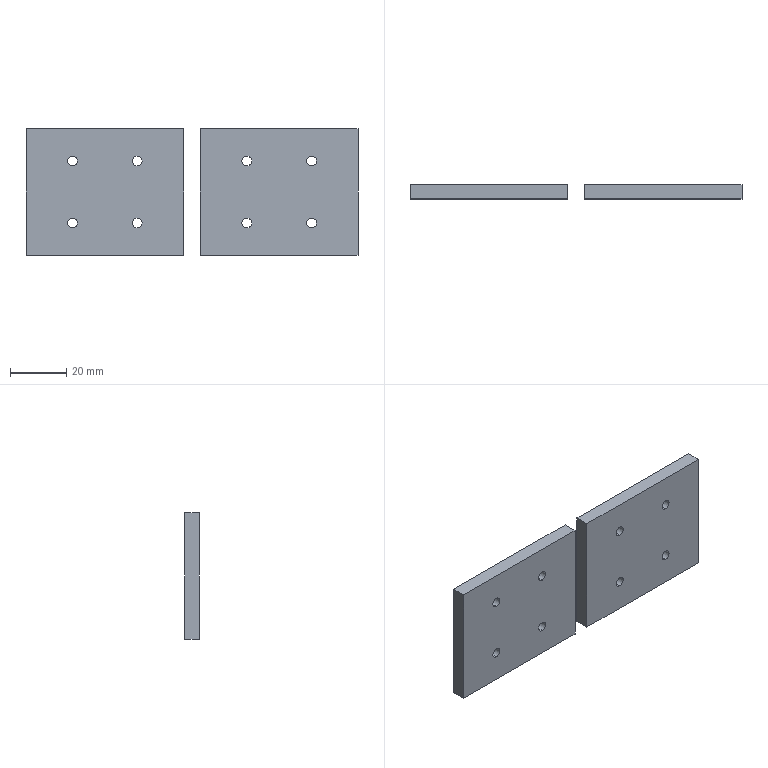CAM job | Mastercam | mm | 4 operations | part box 118 x 5 x 45
1. Contour (Ramp) | 2 - 2 平铣刀
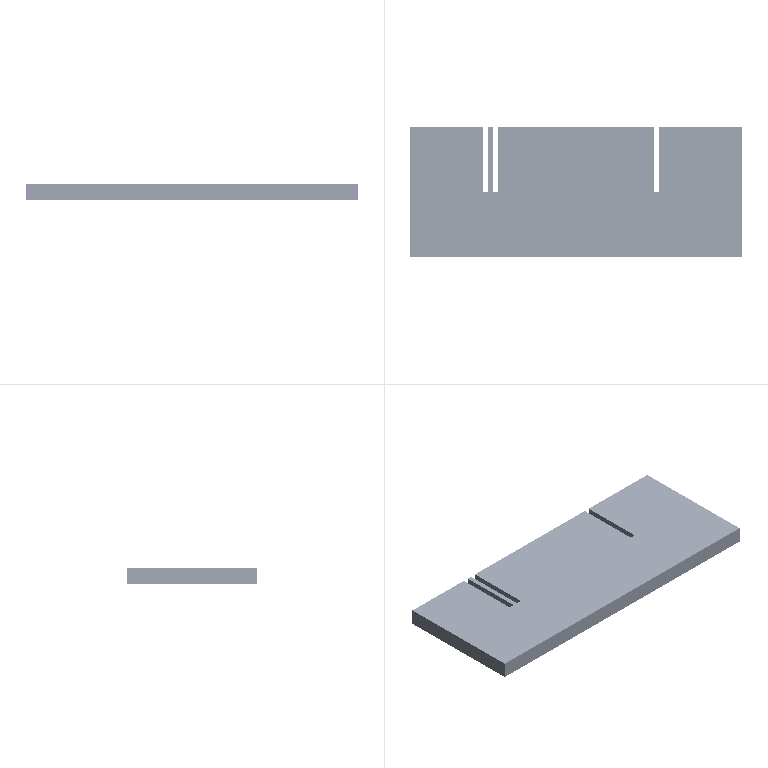2. Contour (2D) | 2 - 2 平铣刀
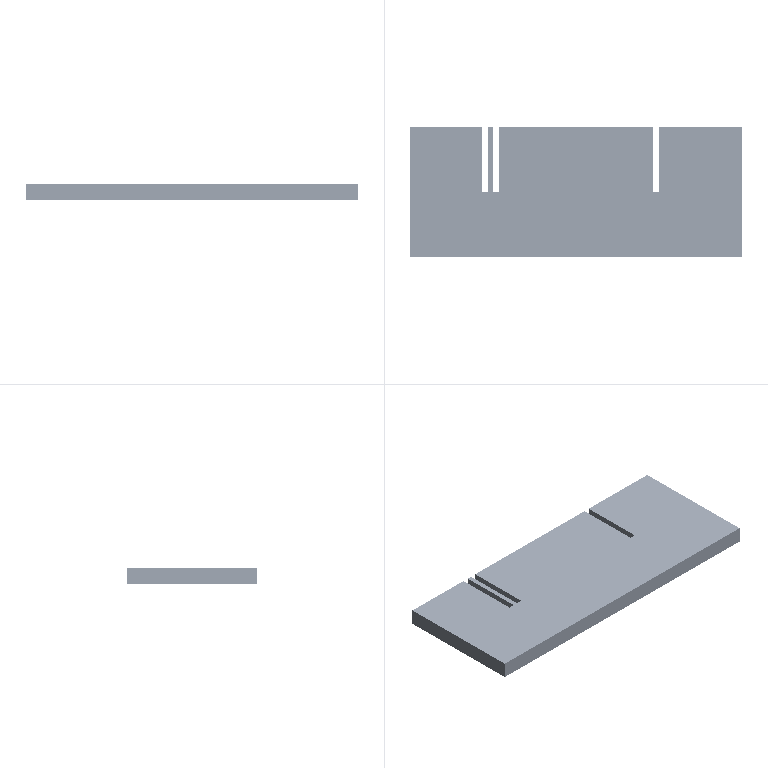3. Drill/Counterbore | 5 - 4 倒角刀
4. Contour (2D chamfer) | 5 - 4 倒角刀